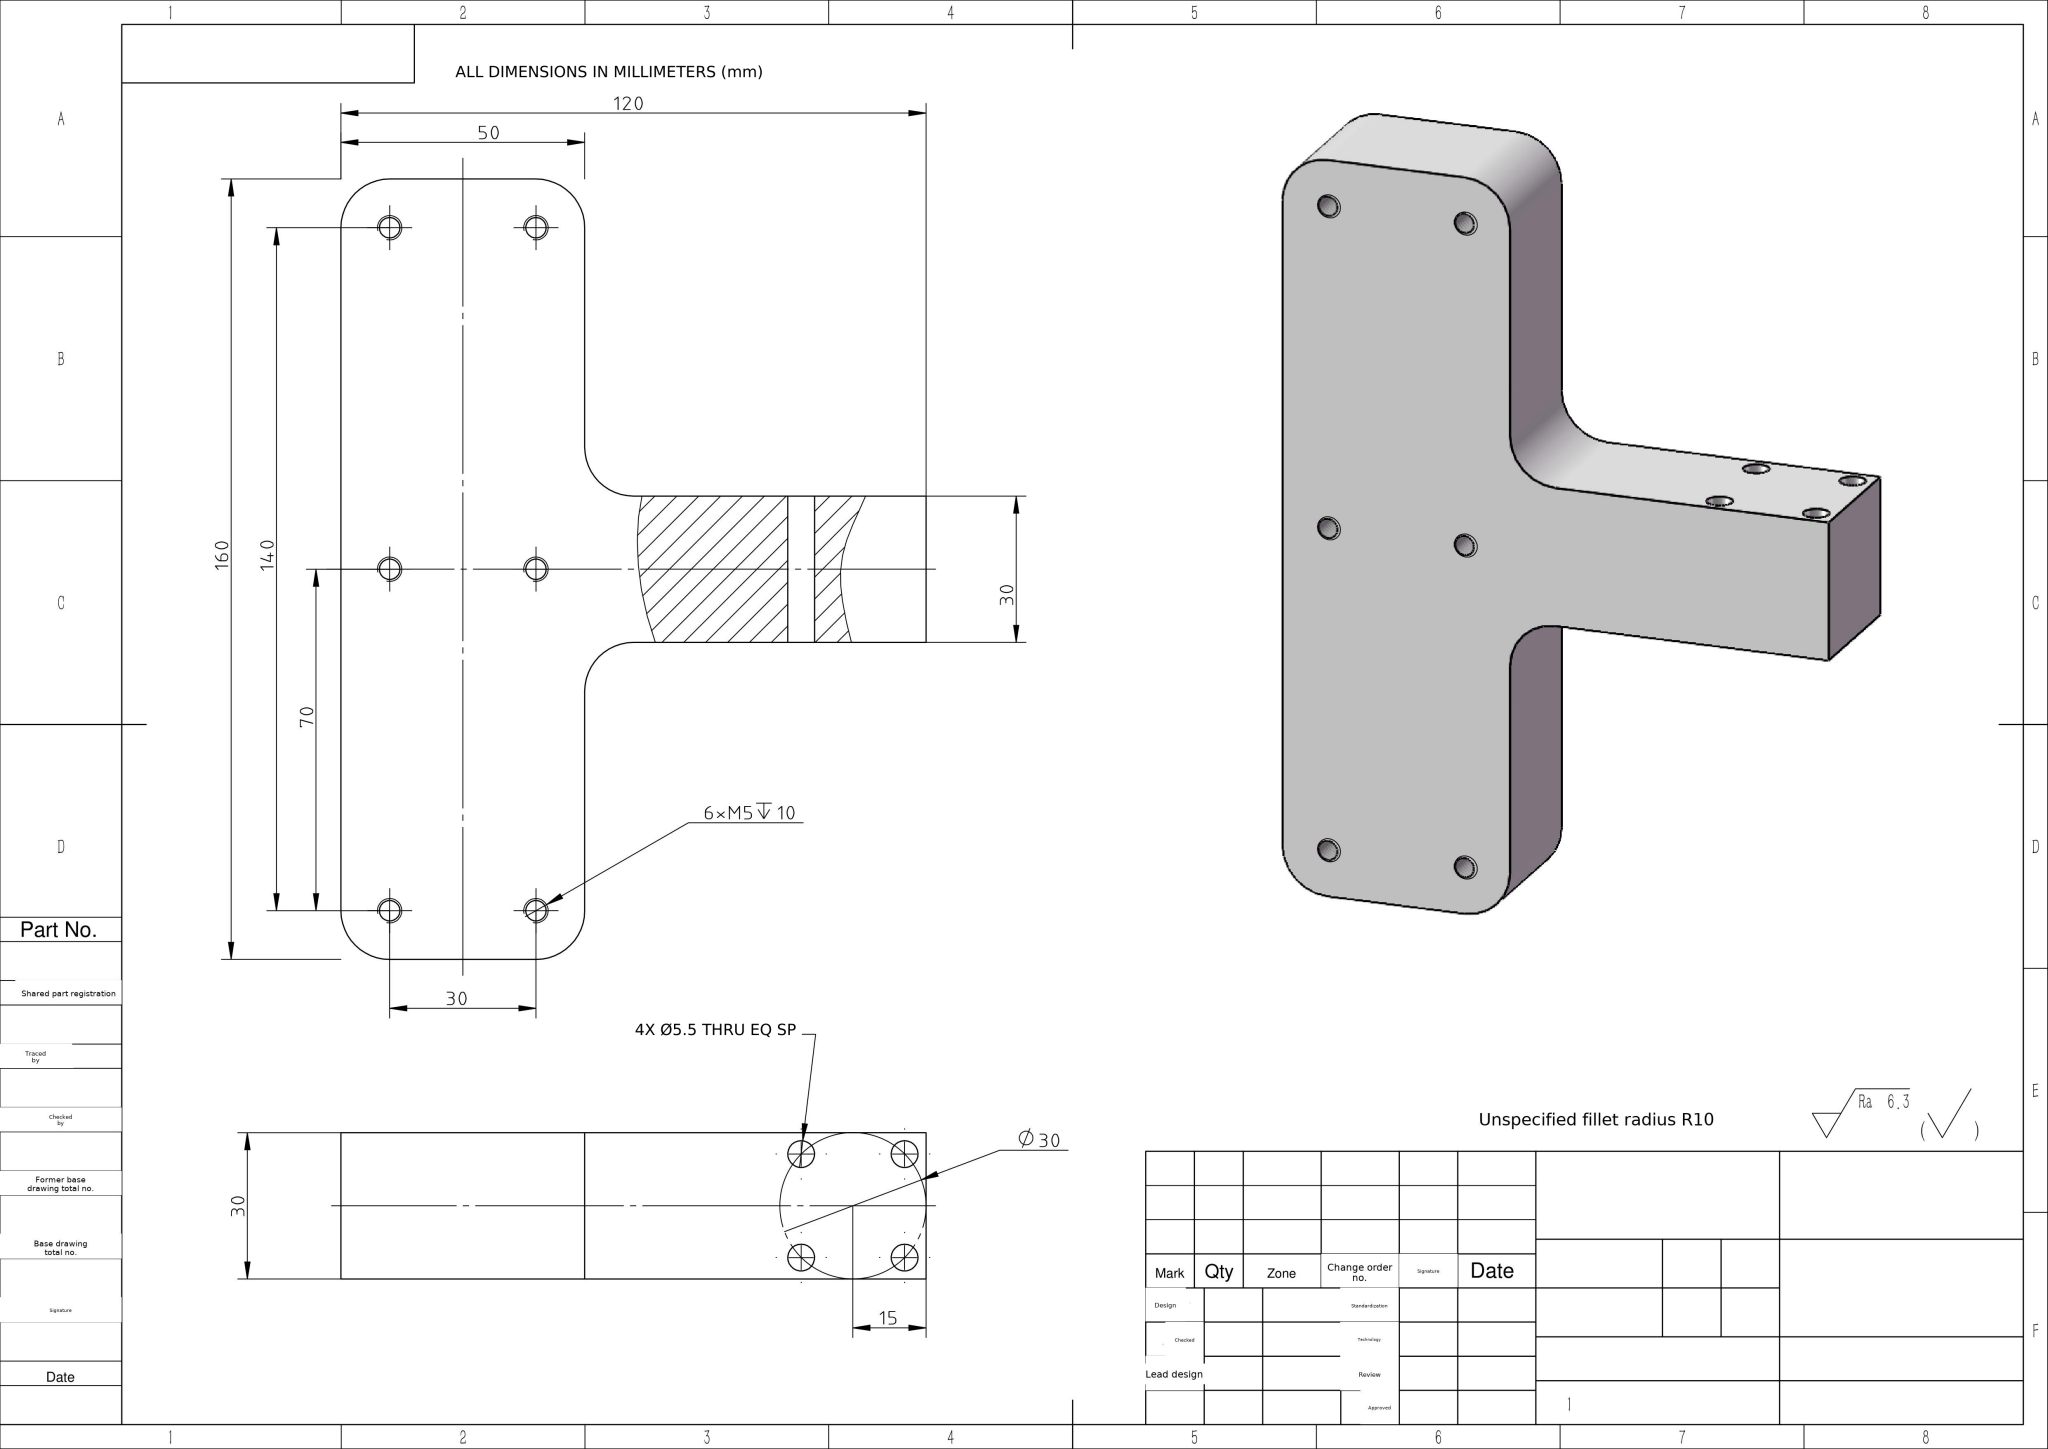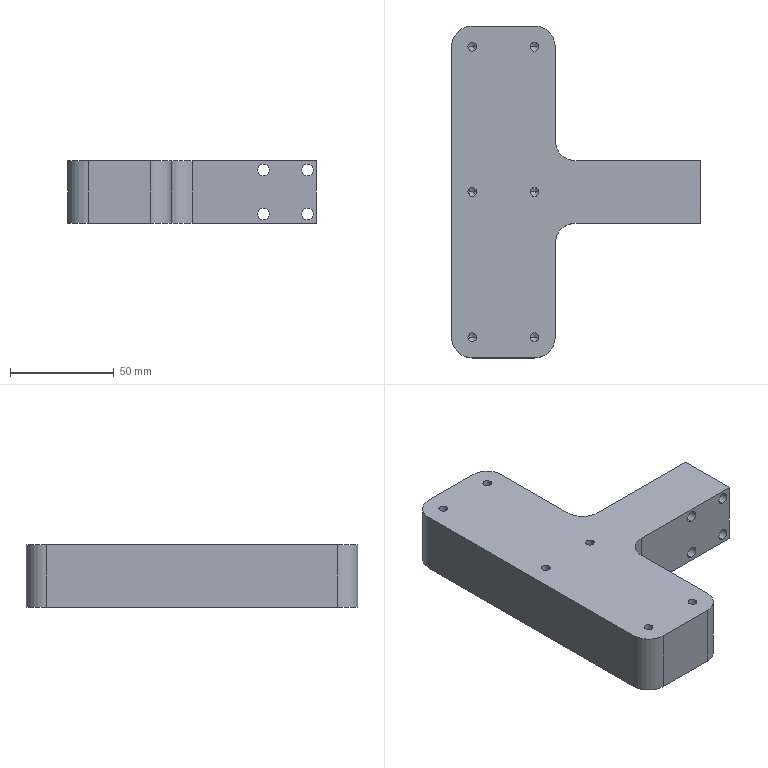Part | NX | mm | 1 solid | 48 faces | box 120 x 160 x 30 mm | volume 297664 mm3 | cylinder 26 | cone 12 | plane 10 | commonest cylinder face diameters 4.2 x12 5.5 x8 20 x6